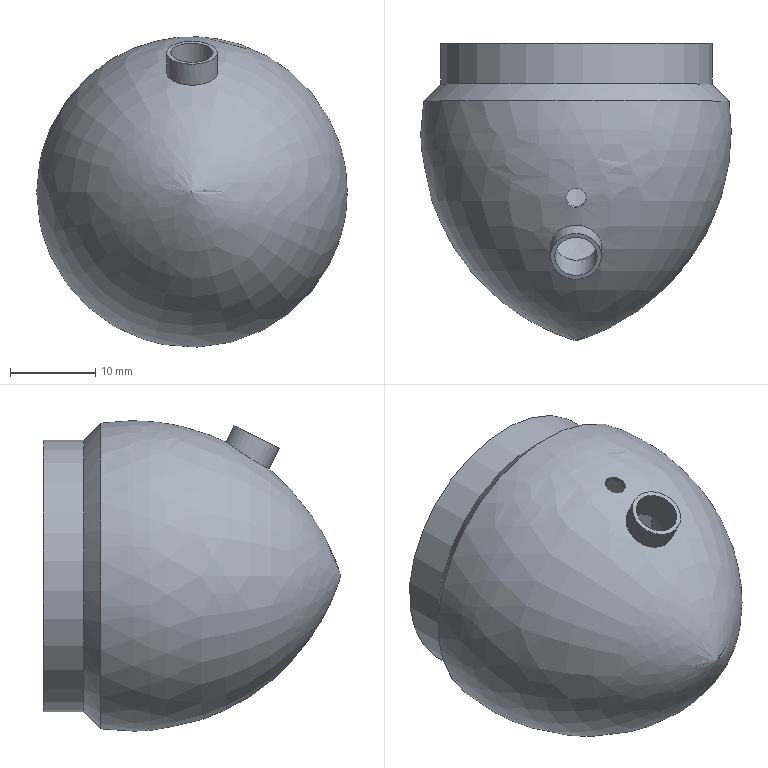Component | NX | CYLINDER_CAP | 1 solid | 13 faces | volume 1745 mm3 | cylinder 6 | plane 3 | spline 2 | cone 2 | commonest cylinder face diameters 6 x2 32 x1 31 x1 5 x1 2.4 x1